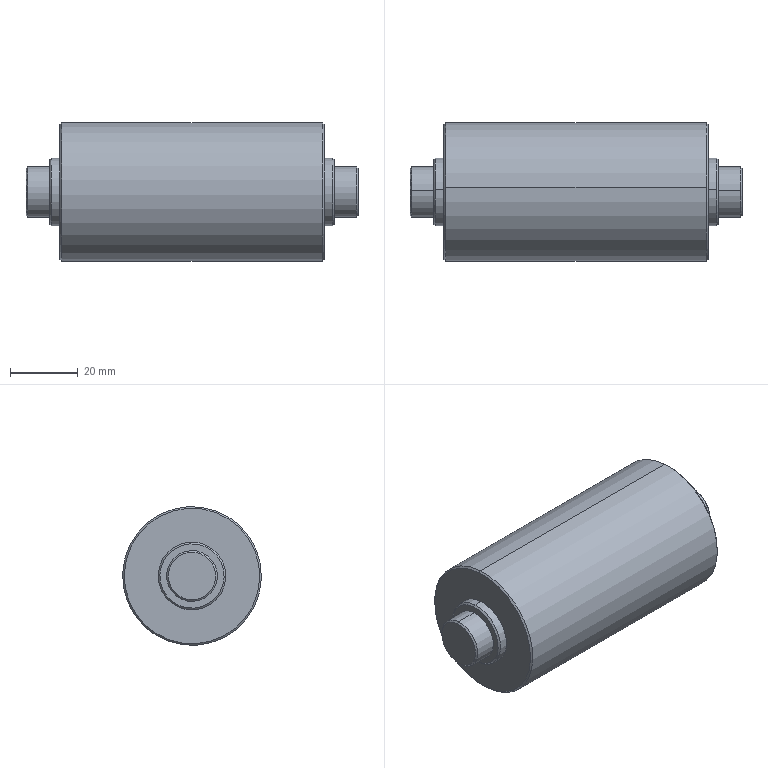Component | SolidWorks | ConveyorDrivenWheel-1 | 1 solid | 28 faces | box 98 x 41 x 41 mm | volume 107280 mm3 | cone 12 | cylinder 10 | plane 6 | commonest cylinder face diameters 15 x4 20 x4 41 x2 | material Plain Carbon Steel
build123d program:
from build123d import *

# Parameters (mm, degrees)
SKETCH1_R           = 20.5
BOSS_EXTRUDE1_DEPTH = 78
SKETCH2_R           = 10
BOSS_EXTRUDE2_DEPTH = 3
BOSS_EXTRUDE3_START = 3
SKETCH3_R           = 10
BOSS_EXTRUDE3_DEPTH = 3
SKETCH4_R           = 7.5
BOSS_EXTRUDE4_DEPTH = 7
BOSS_EXTRUDE5_START = 7
SKETCH5_R           = 7.5
BOSS_EXTRUDE5_DEPTH = 7
CHAMFER1_SIZE       = 0.5


with BuildPart() as part:
    # Sketch1 → Boss-Extrude1 (new body)
    with BuildSketch(Plane.XY):
        Circle(SKETCH1_R)
    extrude(amount=BOSS_EXTRUDE1_DEPTH)

    # Sketch2 → Boss-Extrude2 (add)
    with BuildSketch(Plane.XY.offset(78)):
        Circle(SKETCH2_R)
    extrude(amount=BOSS_EXTRUDE2_DEPTH)

    # Sketch3 → Boss-Extrude3 (add)
    with BuildSketch(Plane(origin=(0, 0, 0), x_dir=(-1, 0, 0), z_dir=(0, 0, -1)).offset(BOSS_EXTRUDE3_START)):
        with Locations(Location((0, 0, 0), (0, 0, 180))):
            Circle(SKETCH3_R)
    extrude(amount=-BOSS_EXTRUDE3_DEPTH)

    # Sketch4 → Boss-Extrude4 (add)
    with BuildSketch(Plane.XY.offset(81)):
        Circle(SKETCH4_R)
    extrude(amount=BOSS_EXTRUDE4_DEPTH)

    # Sketch5 → Boss-Extrude5 (add)
    with BuildSketch(Plane(origin=(0, 0, -3), x_dir=(-1, 0, 0), z_dir=(0, 0, -1)).offset(BOSS_EXTRUDE5_START)):
        with Locations(Location((0, 0, 0), (0, 0, 180))):
            Circle(SKETCH5_R)
    extrude(amount=-BOSS_EXTRUDE5_DEPTH)

    # Chamfer1
    chamfer1_edges = [part.edges().sort_by_distance(p)[0] for p in [
        (-10, 0, -3),
        (-7.5, 0, 88),
        (-20.5, 0, 0),
        (-7.5, 0, -10),
        (-20.5, 0, 78),
        (-10, 0, 81),
    ]]
    chamfer(chamfer1_edges, length=CHAMFER1_SIZE)


solid = part.part

# Placed as in the assembly
solid = solid.moved(Location((-44.55, 5.646, 155), (0, 90, 0)))
STEP:
#1=CARTESIAN_POINT('',(-1.754,0.2749,6.888));
#2=VERTEX_POINT('',#1);
#3=CARTESIAN_POINT('',(-1.754,0.1697,5.317));
#4=VERTEX_POINT('',#3);
#5=CARTESIAN_POINT('',(-1.754,0.2223,6.102));
#6=DIRECTION('',(-1.,0.,0.));
#7=DIRECTION('',(0.,0.06681,0.9978));
#8=AXIS2_PLACEMENT_3D('',#5,#6,#7);
#9=CIRCLE('',#8,0.7874);
#10=EDGE_CURVE('',#2,#4,#9,.T.);
#11=ORIENTED_EDGE('',*,*,#10,.F.);
#12=CARTESIAN_POINT('',(-1.734,0.2762,6.908));
#13=VERTEX_POINT('',#12);
#14=CARTESIAN_POINT('',(-1.754,0.2749,6.888));
#15=DIRECTION('',(0.7071,0.04724,0.7055));
#16=VECTOR('',#15,39.37);
#17=LINE('',#14,#16);
#18=EDGE_CURVE('',#2,#13,#17,.T.);
#19=ORIENTED_EDGE('',*,*,#18,.T.);
#20=CARTESIAN_POINT('',(-1.734,0.1684,5.297));
#21=VERTEX_POINT('',#20);
#22=CARTESIAN_POINT('',(-1.734,0.2223,6.102));
#23=DIRECTION('',(1.,0.,0.));
#24=DIRECTION('',(0.,0.06681,0.9978));
#25=AXIS2_PLACEMENT_3D('',#22,#23,#24);
#26=CIRCLE('',#25,0.8071);
#27=EDGE_CURVE('',#21,#13,#26,.T.);
#28=ORIENTED_EDGE('',*,*,#27,.F.);
#29=CARTESIAN_POINT('',(-1.754,0.1697,5.317));
#30=DIRECTION('',(0.7071,-0.04724,-0.7055));
#31=VECTOR('',#30,39.37);
#32=LINE('',#29,#31);
#33=EDGE_CURVE('',#4,#21,#32,.T.);
#34=ORIENTED_EDGE('',*,*,#33,.F.);
#35=EDGE_LOOP('',(#11,#19,#28,#34));
#36=FACE_OUTER_BOUND('',#35,.T.);
#37=CARTESIAN_POINT('',(-1.754,0.2223,6.102));
#38=DIRECTION('',(1.,0.,0.));
#39=DIRECTION('',(0.,-0.06681,-0.9978));
#40=AXIS2_PLACEMENT_3D('',#37,#38,#39);
#41=CONICAL_SURFACE('',#40,0.7874,0.7854);
#42=ADVANCED_FACE('',(#36),#41,.T.);
#43=CARTESIAN_POINT('',(1.317,0.1697,5.317));
#44=VERTEX_POINT('',#43);
#45=CARTESIAN_POINT('',(1.317,0.2749,6.888));
#46=VERTEX_POINT('',#45);
#47=CARTESIAN_POINT('',(1.317,0.2223,6.102));
#48=DIRECTION('',(1.,0.,0.));
#49=DIRECTION('',(0.,0.06681,0.9978));
#50=AXIS2_PLACEMENT_3D('',#47,#48,#49);
#51=CIRCLE('',#50,0.7874);
#52=EDGE_CURVE('',#44,#46,#51,.T.);
#53=ORIENTED_EDGE('',*,*,#52,.F.);
#54=CARTESIAN_POINT('',(1.297,0.1684,5.297));
#55=VERTEX_POINT('',#54);
#56=CARTESIAN_POINT('',(1.297,0.1684,5.297));
#57=DIRECTION('',(-0.7071,-0.04724,-0.7055));
#58=VECTOR('',#57,39.37);
#59=LINE('',#56,#58);
#60=EDGE_CURVE('',#44,#55,#59,.T.);
#61=ORIENTED_EDGE('',*,*,#60,.T.);
#62=CARTESIAN_POINT('',(1.297,0.2762,6.908));
#63=VERTEX_POINT('',#62);
#64=CARTESIAN_POINT('',(1.297,0.2223,6.102));
#65=DIRECTION('',(-1.,0.,0.));
#66=DIRECTION('',(0.,0.06681,0.9978));
#67=AXIS2_PLACEMENT_3D('',#64,#65,#66);
#68=CIRCLE('',#67,0.8071);
#69=EDGE_CURVE('',#63,#55,#68,.T.);
#70=ORIENTED_EDGE('',*,*,#69,.F.);
#71=CARTESIAN_POINT('',(1.297,0.2762,6.908));
#72=DIRECTION('',(-0.7071,0.04724,0.7055));
#73=VECTOR('',#72,39.37);
#74=LINE('',#71,#73);
#75=EDGE_CURVE('',#46,#63,#74,.T.);
#76=ORIENTED_EDGE('',*,*,#75,.F.);
#77=EDGE_LOOP('',(#53,#61,#70,#76));
#78=FACE_OUTER_BOUND('',#77,.T.);
#79=CARTESIAN_POINT('',(1.297,0.2223,6.102));
#80=DIRECTION('',(-1.,0.,0.));
#81=DIRECTION('',(0.,0.06681,0.9978));
#82=AXIS2_PLACEMENT_3D('',#79,#80,#81);
#83=CONICAL_SURFACE('',#82,0.8071,0.7854);
#84=ADVANCED_FACE('',(#78),#83,.T.);
#85=CARTESIAN_POINT('',(-2.148,0.2407,6.377));
#86=VERTEX_POINT('',#85);
#87=CARTESIAN_POINT('',(-2.148,0.2039,5.827));
#88=VERTEX_POINT('',#87);
#89=CARTESIAN_POINT('',(-2.148,0.2223,6.102));
#90=DIRECTION('',(-1.,0.,0.));
#91=DIRECTION('',(0.,0.06681,0.9978));
#92=AXIS2_PLACEMENT_3D('',#89,#90,#91);
#93=CIRCLE('',#92,0.2756);
#94=EDGE_CURVE('',#86,#88,#93,.T.);
#95=ORIENTED_EDGE('',*,*,#94,.F.);
#96=CARTESIAN_POINT('',(-2.128,0.242,6.397));
#97=VERTEX_POINT('',#96);
#98=CARTESIAN_POINT('',(-2.148,0.2407,6.377));
#99=DIRECTION('',(0.7071,0.04724,0.7055));
#100=VECTOR('',#99,39.37);
#101=LINE('',#98,#100);
#102=EDGE_CURVE('',#86,#97,#101,.T.);
#103=ORIENTED_EDGE('',*,*,#102,.T.);
#104=CARTESIAN_POINT('',(-2.128,0.2025,5.808));
#105=VERTEX_POINT('',#104);
#106=CARTESIAN_POINT('',(-2.128,0.2223,6.102));
#107=DIRECTION('',(1.,0.,0.));
#108=DIRECTION('',(0.,0.06681,0.9978));
#109=AXIS2_PLACEMENT_3D('',#106,#107,#108);
#110=CIRCLE('',#109,0.2953);
#111=EDGE_CURVE('',#105,#97,#110,.T.);
#112=ORIENTED_EDGE('',*,*,#111,.F.);
#113=CARTESIAN_POINT('',(-2.148,0.2039,5.827));
#114=DIRECTION('',(0.7071,-0.04724,-0.7055));
#115=VECTOR('',#114,39.37);
#116=LINE('',#113,#115);
#117=EDGE_CURVE('',#88,#105,#116,.T.);
#118=ORIENTED_EDGE('',*,*,#117,.F.);
#119=EDGE_LOOP('',(#95,#103,#112,#118));
#120=FACE_OUTER_BOUND('',#119,.T.);
#121=CARTESIAN_POINT('',(-2.148,0.2223,6.102));
#122=DIRECTION('',(1.,0.,0.));
#123=DIRECTION('',(0.,-0.06681,-0.9978));
#124=AXIS2_PLACEMENT_3D('',#121,#122,#123);
#125=CONICAL_SURFACE('',#124,0.2756,0.7854);
#126=ADVANCED_FACE('',(#120),#125,.T.);
#127=CARTESIAN_POINT('',(-1.872,0.2473,6.476));
#128=VERTEX_POINT('',#127);
#129=CARTESIAN_POINT('',(-1.872,0.1973,5.729));
#130=VERTEX_POINT('',#129);
#131=CARTESIAN_POINT('',(-1.872,0.2223,6.102));
#132=DIRECTION('',(-1.,0.,0.));
#133=DIRECTION('',(0.,0.06681,0.9978));
#134=AXIS2_PLACEMENT_3D('',#131,#132,#133);
#135=CIRCLE('',#134,0.374);
#136=EDGE_CURVE('',#128,#130,#135,.T.);
#137=ORIENTED_EDGE('',*,*,#136,.F.);
#138=CARTESIAN_POINT('',(-1.852,0.2486,6.495));
#139=VERTEX_POINT('',#138);
#140=CARTESIAN_POINT('',(-1.872,0.2473,6.476));
#141=DIRECTION('',(0.7071,0.04724,0.7055));
#142=VECTOR('',#141,39.37);
#143=LINE('',#140,#142);
#144=EDGE_CURVE('',#128,#139,#143,.T.);
#145=ORIENTED_EDGE('',*,*,#144,.T.);
#146=CARTESIAN_POINT('',(-1.852,0.196,5.71));
#147=VERTEX_POINT('',#146);
#148=CARTESIAN_POINT('',(-1.852,0.2223,6.102));
#149=DIRECTION('',(1.,0.,0.));
#150=DIRECTION('',(0.,0.06681,0.9978));
#151=AXIS2_PLACEMENT_3D('',#148,#149,#150);
#152=CIRCLE('',#151,0.3937);
#153=EDGE_CURVE('',#147,#139,#152,.T.);
#154=ORIENTED_EDGE('',*,*,#153,.F.);
#155=CARTESIAN_POINT('',(-1.872,0.1973,5.729));
#156=DIRECTION('',(0.7071,-0.04724,-0.7055));
#157=VECTOR('',#156,39.37);
#158=LINE('',#155,#157);
#159=EDGE_CURVE('',#130,#147,#158,.T.);
#160=ORIENTED_EDGE('',*,*,#159,.F.);
#161=EDGE_LOOP('',(#137,#145,#154,#160));
#162=FACE_OUTER_BOUND('',#161,.T.);
#163=CARTESIAN_POINT('',(-1.872,0.2223,6.102));
#164=DIRECTION('',(1.,0.,0.));
#165=DIRECTION('',(0.,-0.06681,-0.9978));
#166=AXIS2_PLACEMENT_3D('',#163,#164,#165);
#167=CONICAL_SURFACE('',#166,0.374,0.7854);
#168=ADVANCED_FACE('',(#162),#167,.T.);
#169=CARTESIAN_POINT('',(1.435,0.1973,5.729));
#170=VERTEX_POINT('',#169);
#171=CARTESIAN_POINT('',(1.435,0.2473,6.476));
#172=VERTEX_POINT('',#171);
#173=CARTESIAN_POINT('',(1.435,0.2223,6.102));
#174=DIRECTION('',(1.,0.,0.));
#175=DIRECTION('',(0.,-0.06681,-0.9978));
#176=AXIS2_PLACEMENT_3D('',#173,#174,#175);
#177=CIRCLE('',#176,0.374);
#178=EDGE_CURVE('',#170,#172,#177,.T.);
#179=ORIENTED_EDGE('',*,*,#178,.F.);
#180=CARTESIAN_POINT('',(1.415,0.196,5.71));
#181=VERTEX_POINT('',#180);
#182=CARTESIAN_POINT('',(1.435,0.1973,5.729));
#183=DIRECTION('',(-0.7071,-0.04724,-0.7055));
#184=VECTOR('',#183,39.37);
#185=LINE('',#182,#184);
#186=EDGE_CURVE('',#170,#181,#185,.T.);
#187=ORIENTED_EDGE('',*,*,#186,.T.);
#188=CARTESIAN_POINT('',(1.415,0.2486,6.495));
#189=VERTEX_POINT('',#188);
#190=CARTESIAN_POINT('',(1.415,0.2223,6.102));
#191=DIRECTION('',(-1.,0.,0.));
#192=DIRECTION('',(0.,-0.06681,-0.9978));
#193=AXIS2_PLACEMENT_3D('',#190,#191,#192);
#194=CIRCLE('',#193,0.3937);
#195=EDGE_CURVE('',#189,#181,#194,.T.);
#196=ORIENTED_EDGE('',*,*,#195,.F.);
#197=CARTESIAN_POINT('',(1.435,0.2473,6.476));
#198=DIRECTION('',(-0.7071,0.04724,0.7055));
#199=VECTOR('',#198,39.37);
#200=LINE('',#197,#199);
#201=EDGE_CURVE('',#172,#189,#200,.T.);
#202=ORIENTED_EDGE('',*,*,#201,.F.);
#203=EDGE_LOOP('',(#179,#187,#196,#202));
#204=FACE_OUTER_BOUND('',#203,.T.);
#205=CARTESIAN_POINT('',(1.435,0.2223,6.102));
#206=DIRECTION('',(-1.,0.,0.));
#207=DIRECTION('',(0.,0.06681,0.9978));
#208=AXIS2_PLACEMENT_3D('',#205,#206,#207);
#209=CONICAL_SURFACE('',#208,0.374,0.7854);
#210=ADVANCED_FACE('',(#204),#209,.T.);
#211=CARTESIAN_POINT('',(1.711,0.2039,5.827));
#212=VERTEX_POINT('',#211);
#213=CARTESIAN_POINT('',(1.711,0.2407,6.377));
#214=VERTEX_POINT('',#213);
#215=CARTESIAN_POINT('',(1.711,0.2223,6.102));
#216=DIRECTION('',(1.,0.,0.));
#217=DIRECTION('',(0.,-0.06681,-0.9978));
#218=AXIS2_PLACEMENT_3D('',#215,#216,#217);
#219=CIRCLE('',#218,0.2756);
#220=EDGE_CURVE('',#212,#214,#219,.T.);
#221=ORIENTED_EDGE('',*,*,#220,.F.);
#222=CARTESIAN_POINT('',(1.691,0.2025,5.808));
#223=VERTEX_POINT('',#222);
#224=CARTESIAN_POINT('',(1.711,0.2039,5.827));
#225=DIRECTION('',(-0.7071,-0.04724,-0.7055));
#226=VECTOR('',#225,39.37);
#227=LINE('',#224,#226);
#228=EDGE_CURVE('',#212,#223,#227,.T.);
#229=ORIENTED_EDGE('',*,*,#228,.T.);
#230=CARTESIAN_POINT('',(1.691,0.242,6.397));
#231=VERTEX_POINT('',#230);
#232=CARTESIAN_POINT('',(1.691,0.2223,6.102));
#233=DIRECTION('',(-1.,0.,0.));
#234=DIRECTION('',(0.,-0.06681,-0.9978));
#235=AXIS2_PLACEMENT_3D('',#232,#233,#234);
#236=CIRCLE('',#235,0.2953);
#237=EDGE_CURVE('',#231,#223,#236,.T.);
#238=ORIENTED_EDGE('',*,*,#237,.F.);
#239=CARTESIAN_POINT('',(1.711,0.2407,6.377));
#240=DIRECTION('',(-0.7071,0.04724,0.7055));
#241=VECTOR('',#240,39.37);
#242=LINE('',#239,#241);
#243=EDGE_CURVE('',#214,#231,#242,.T.);
#244=ORIENTED_EDGE('',*,*,#243,.F.);
#245=EDGE_LOOP('',(#221,#229,#238,#244));
#246=FACE_OUTER_BOUND('',#245,.T.);
#247=CARTESIAN_POINT('',(1.711,0.2223,6.102));
#248=DIRECTION('',(-1.,0.,0.));
#249=DIRECTION('',(0.,0.06681,0.9978));
#250=AXIS2_PLACEMENT_3D('',#247,#248,#249);
#251=CONICAL_SURFACE('',#250,0.2756,0.7854);
#252=ADVANCED_FACE('',(#246),#251,.T.);
#253=ORIENTED_EDGE('',*,*,#237,.T.);
#254=CARTESIAN_POINT('',(1.435,0.2025,5.808));
#255=VERTEX_POINT('',#254);
#256=CARTESIAN_POINT('',(1.711,0.2025,5.808));
#257=DIRECTION('',(-1.,0.,0.));
#258=VECTOR('',#257,39.37);
#259=LINE('',#256,#258);
#260=EDGE_CURVE('',#223,#255,#259,.T.);
#261=ORIENTED_EDGE('',*,*,#260,.T.);
#262=CARTESIAN_POINT('',(1.435,0.242,6.397));
#263=VERTEX_POINT('',#262);
#264=CARTESIAN_POINT('',(1.435,0.2223,6.102));
#265=DIRECTION('',(1.,0.,0.));
#266=DIRECTION('',(0.,-0.06681,-0.9978));
#267=AXIS2_PLACEMENT_3D('',#264,#265,#266);
#268=CIRCLE('',#267,0.2953);
#269=EDGE_CURVE('',#255,#263,#268,.T.);
#270=ORIENTED_EDGE('',*,*,#269,.T.);
#271=CARTESIAN_POINT('',(1.711,0.242,6.397));
#272=DIRECTION('',(-1.,0.,0.));
#273=VECTOR('',#272,39.37);
#274=LINE('',#271,#273);
#275=EDGE_CURVE('',#231,#263,#274,.T.);
#276=ORIENTED_EDGE('',*,*,#275,.F.);
#277=EDGE_LOOP('',(#253,#261,#270,#276));
#278=FACE_OUTER_BOUND('',#277,.T.);
#279=CARTESIAN_POINT('',(1.711,0.2223,6.102));
#280=DIRECTION('',(-1.,0.,0.));
#281=DIRECTION('',(0.,0.06681,0.9978));
#282=AXIS2_PLACEMENT_3D('',#279,#280,#281);
#283=CYLINDRICAL_SURFACE('',#282,0.2953);
#284=ADVANCED_FACE('',(#278),#283,.T.);
#285=ORIENTED_EDGE('',*,*,#111,.T.);
#286=CARTESIAN_POINT('',(-1.872,0.242,6.397));
#287=VERTEX_POINT('',#286);
#288=CARTESIAN_POINT('',(-2.148,0.242,6.397));
#289=DIRECTION('',(1.,0.,0.));
#290=VECTOR('',#289,39.37);
#291=LINE('',#288,#290);
#292=EDGE_CURVE('',#97,#287,#291,.T.);
#293=ORIENTED_EDGE('',*,*,#292,.T.);
#294=CARTESIAN_POINT('',(-1.872,0.2025,5.808));
#295=VERTEX_POINT('',#294);
#296=CARTESIAN_POINT('',(-1.872,0.2223,6.102));
#297=DIRECTION('',(-1.,0.,0.));
#298=DIRECTION('',(0.,0.06681,0.9978));
#299=AXIS2_PLACEMENT_3D('',#296,#297,#298);
#300=CIRCLE('',#299,0.2953);
#301=EDGE_CURVE('',#287,#295,#300,.T.);
#302=ORIENTED_EDGE('',*,*,#301,.T.);
#303=CARTESIAN_POINT('',(-2.148,0.2025,5.808));
#304=DIRECTION('',(1.,0.,0.));
#305=VECTOR('',#304,39.37);
#306=LINE('',#303,#305);
#307=EDGE_CURVE('',#105,#295,#306,.T.);
#308=ORIENTED_EDGE('',*,*,#307,.F.);
#309=EDGE_LOOP('',(#285,#293,#302,#308));
#310=FACE_OUTER_BOUND('',#309,.T.);
#311=CARTESIAN_POINT('',(-2.148,0.2223,6.102));
#312=DIRECTION('',(1.,0.,0.));
#313=DIRECTION('',(0.,-0.06681,-0.9978));
#314=AXIS2_PLACEMENT_3D('',#311,#312,#313);
#315=CYLINDRICAL_SURFACE('',#314,0.2953);
#316=ADVANCED_FACE('',(#310),#315,.T.);
#317=ORIENTED_EDGE('',*,*,#195,.T.);
#318=CARTESIAN_POINT('',(1.317,0.196,5.71));
#319=VERTEX_POINT('',#318);
#320=CARTESIAN_POINT('',(1.435,0.196,5.71));
#321=DIRECTION('',(-1.,0.,0.));
#322=VECTOR('',#321,39.37);
#323=LINE('',#320,#322);
#324=EDGE_CURVE('',#181,#319,#323,.T.);
#325=ORIENTED_EDGE('',*,*,#324,.T.);
#326=CARTESIAN_POINT('',(1.317,0.2486,6.495));
#327=VERTEX_POINT('',#326);
#328=CARTESIAN_POINT('',(1.317,0.2223,6.102));
#329=DIRECTION('',(1.,0.,0.));
#330=DIRECTION('',(0.,0.06681,0.9978));
#331=AXIS2_PLACEMENT_3D('',#328,#329,#330);
#332=CIRCLE('',#331,0.3937);
#333=EDGE_CURVE('',#319,#327,#332,.T.);
#334=ORIENTED_EDGE('',*,*,#333,.T.);
#335=CARTESIAN_POINT('',(1.435,0.2486,6.495));
#336=DIRECTION('',(-1.,0.,0.));
#337=VECTOR('',#336,39.37);
#338=LINE('',#335,#337);
#339=EDGE_CURVE('',#189,#327,#338,.T.);
#340=ORIENTED_EDGE('',*,*,#339,.F.);
#341=EDGE_LOOP('',(#317,#325,#334,#340));
#342=FACE_OUTER_BOUND('',#341,.T.);
#343=CARTESIAN_POINT('',(1.435,0.2223,6.102));
#344=DIRECTION('',(-1.,0.,0.));
#345=DIRECTION('',(0.,0.06681,0.9978));
#346=AXIS2_PLACEMENT_3D('',#343,#344,#345);
#347=CYLINDRICAL_SURFACE('',#346,0.3937);
#348=ADVANCED_FACE('',(#342),#347,.T.);
#349=ORIENTED_EDGE('',*,*,#153,.T.);
#350=CARTESIAN_POINT('',(-1.754,0.2486,6.495));
#351=VERTEX_POINT('',#350);
#352=CARTESIAN_POINT('',(-1.872,0.2486,6.495));
#353=DIRECTION('',(1.,0.,0.));
#354=VECTOR('',#353,39.37);
#355=LINE('',#352,#354);
#356=EDGE_CURVE('',#139,#351,#355,.T.);
#357=ORIENTED_EDGE('',*,*,#356,.T.);
#358=CARTESIAN_POINT('',(-1.754,0.196,5.71));
#359=VERTEX_POINT('',#358);
#360=CARTESIAN_POINT('',(-1.754,0.2223,6.102));
#361=DIRECTION('',(-1.,0.,0.));
#362=DIRECTION('',(0.,0.06681,0.9978));
#363=AXIS2_PLACEMENT_3D('',#360,#361,#362);
#364=CIRCLE('',#363,0.3937);
#365=EDGE_CURVE('',#351,#359,#364,.T.);
#366=ORIENTED_EDGE('',*,*,#365,.T.);
#367=CARTESIAN_POINT('',(-1.872,0.196,5.71));
#368=DIRECTION('',(1.,0.,0.));
#369=VECTOR('',#368,39.37);
#370=LINE('',#367,#369);
#371=EDGE_CURVE('',#147,#359,#370,.T.);
#372=ORIENTED_EDGE('',*,*,#371,.F.);
#373=EDGE_LOOP('',(#349,#357,#366,#372));
#374=FACE_OUTER_BOUND('',#373,.T.);
#375=CARTESIAN_POINT('',(-1.872,0.2223,6.102));
#376=DIRECTION('',(1.,0.,0.));
#377=DIRECTION('',(0.,-0.06681,-0.9978));
#378=AXIS2_PLACEMENT_3D('',#375,#376,#377);
#379=CYLINDRICAL_SURFACE('',#378,0.3937);
#380=ADVANCED_FACE('',(#374),#379,.T.);
#381=ORIENTED_EDGE('',*,*,#27,.T.);
#382=CARTESIAN_POINT('',(-1.754,0.2762,6.908));
#383=DIRECTION('',(1.,0.,0.));
#384=VECTOR('',#383,39.37);
#385=LINE('',#382,#384);
#386=EDGE_CURVE('',#13,#63,#385,.T.);
#387=ORIENTED_EDGE('',*,*,#386,.T.);
#388=ORIENTED_EDGE('',*,*,#69,.T.);
#389=CARTESIAN_POINT('',(-1.754,0.1684,5.297));
#390=DIRECTION('',(1.,0.,0.));
#391=VECTOR('',#390,39.37);
#392=LINE('',#389,#391);
#393=EDGE_CURVE('',#21,#55,#392,.T.);
#394=ORIENTED_EDGE('',*,*,#393,.F.);
#395=EDGE_LOOP('',(#381,#387,#388,#394));
#396=FACE_OUTER_BOUND('',#395,.T.);
#397=CARTESIAN_POINT('',(-1.754,0.2223,6.102));
#398=DIRECTION('',(1.,0.,0.));
#399=DIRECTION('',(0.,-0.06681,-0.9978));
#400=AXIS2_PLACEMENT_3D('',#397,#398,#399);
#401=CYLINDRICAL_SURFACE('',#400,0.8071);
#402=ADVANCED_FACE('',(#396),#401,.T.);
#403=CARTESIAN_POINT('',(1.435,0.2223,6.102));
#404=DIRECTION('',(1.,0.,0.));
#405=DIRECTION('',(0.,-0.06681,-0.9978));
#406=AXIS2_PLACEMENT_3D('',#403,#404,#405);
#407=CIRCLE('',#406,0.374);
#408=EDGE_CURVE('',#172,#170,#407,.T.);
#409=ORIENTED_EDGE('',*,*,#408,.T.);
#410=ORIENTED_EDGE('',*,*,#178,.T.);
#411=EDGE_LOOP('',(#409,#410));
#412=FACE_OUTER_BOUND('',#411,.T.);
#413=CARTESIAN_POINT('',(1.435,0.2223,6.102));
#414=DIRECTION('',(1.,0.,0.));
#415=DIRECTION('',(0.,-0.06681,-0.9978));
#416=AXIS2_PLACEMENT_3D('',#413,#414,#415);
#417=CIRCLE('',#416,0.2953);
#418=EDGE_CURVE('',#263,#255,#417,.T.);
#419=ORIENTED_EDGE('',*,*,#418,.F.);
#420=ORIENTED_EDGE('',*,*,#269,.F.);
#421=EDGE_LOOP('',(#419,#420));
#422=FACE_BOUND('',#421,.T.);
#423=CARTESIAN_POINT('',(1.435,0.2223,6.102));
#424=DIRECTION('',(1.,0.,0.));
#425=DIRECTION('',(0.,-0.06681,-0.9978));
#426=AXIS2_PLACEMENT_3D('',#423,#424,#425);
#427=PLANE('',#426);
#428=ADVANCED_FACE('',(#412,#422),#427,.T.);
#429=CARTESIAN_POINT('',(-1.872,0.2223,6.102));
#430=DIRECTION('',(-1.,0.,0.));
#431=DIRECTION('',(0.,0.06681,0.9978));
#432=AXIS2_PLACEMENT_3D('',#429,#430,#431);
#433=CIRCLE('',#432,0.374);
#434=EDGE_CURVE('',#130,#128,#433,.T.);
#435=ORIENTED_EDGE('',*,*,#434,.T.);
#436=ORIENTED_EDGE('',*,*,#136,.T.);
#437=EDGE_LOOP('',(#435,#436));
#438=FACE_OUTER_BOUND('',#437,.T.);
#439=CARTESIAN_POINT('',(-1.872,0.2223,6.102));
#440=DIRECTION('',(-1.,0.,0.));
#441=DIRECTION('',(0.,0.06681,0.9978));
#442=AXIS2_PLACEMENT_3D('',#439,#440,#441);
#443=CIRCLE('',#442,0.2953);
#444=EDGE_CURVE('',#295,#287,#443,.T.);
#445=ORIENTED_EDGE('',*,*,#444,.F.);
#446=ORIENTED_EDGE('',*,*,#301,.F.);
#447=EDGE_LOOP('',(#445,#446));
#448=FACE_BOUND('',#447,.T.);
#449=CARTESIAN_POINT('',(-1.872,0.2223,6.102));
#450=DIRECTION('',(-1.,0.,0.));
#451=DIRECTION('',(0.,0.06681,0.9978));
#452=AXIS2_PLACEMENT_3D('',#449,#450,#451);
#453=PLANE('',#452);
#454=ADVANCED_FACE('',(#438,#448),#453,.T.);
#455=CARTESIAN_POINT('',(1.317,0.2223,6.102));
#456=DIRECTION('',(1.,0.,0.));
#457=DIRECTION('',(0.,0.06681,0.9978));
#458=AXIS2_PLACEMENT_3D('',#455,#456,#457);
#459=CIRCLE('',#458,0.7874);
#460=EDGE_CURVE('',#46,#44,#459,.T.);
#461=ORIENTED_EDGE('',*,*,#460,.T.);
#462=ORIENTED_EDGE('',*,*,#52,.T.);
#463=EDGE_LOOP('',(#461,#462));
#464=FACE_OUTER_BOUND('',#463,.T.);
#465=CARTESIAN_POINT('',(1.317,0.2223,6.102));
#466=DIRECTION('',(1.,0.,0.));
#467=DIRECTION('',(0.,0.06681,0.9978));
#468=AXIS2_PLACEMENT_3D('',#465,#466,#467);
#469=CIRCLE('',#468,0.3937);
#470=EDGE_CURVE('',#327,#319,#469,.T.);
#471=ORIENTED_EDGE('',*,*,#470,.F.);
#472=ORIENTED_EDGE('',*,*,#333,.F.);
#473=EDGE_LOOP('',(#471,#472));
#474=FACE_BOUND('',#473,.T.);
#475=CARTESIAN_POINT('',(1.317,0.2223,6.102));
#476=DIRECTION('',(-1.,0.,0.));
#477=DIRECTION('',(0.,0.06681,0.9978));
#478=AXIS2_PLACEMENT_3D('',#475,#476,#477);
#479=PLANE('',#478);
#480=ADVANCED_FACE('',(#464,#474),#479,.F.);
#481=CARTESIAN_POINT('',(-1.754,0.2223,6.102));
#482=DIRECTION('',(-1.,0.,0.));
#483=DIRECTION('',(0.,0.06681,0.9978));
#484=AXIS2_PLACEMENT_3D('',#481,#482,#483);
#485=CIRCLE('',#484,0.7874);
#486=EDGE_CURVE('',#4,#2,#485,.T.);
#487=ORIENTED_EDGE('',*,*,#486,.T.);
#488=ORIENTED_EDGE('',*,*,#10,.T.);
#489=EDGE_LOOP('',(#487,#488));
#490=FACE_OUTER_BOUND('',#489,.T.);
#491=CARTESIAN_POINT('',(-1.754,0.2223,6.102));
#492=DIRECTION('',(-1.,0.,0.));
#493=DIRECTION('',(0.,0.06681,0.9978));
#494=AXIS2_PLACEMENT_3D('',#491,#492,#493);
#495=CIRCLE('',#494,0.3937);
#496=EDGE_CURVE('',#359,#351,#495,.T.);
#497=ORIENTED_EDGE('',*,*,#496,.F.);
#498=ORIENTED_EDGE('',*,*,#365,.F.);
#499=EDGE_LOOP('',(#497,#498));
#500=FACE_BOUND('',#499,.T.);
#501=CARTESIAN_POINT('',(-1.754,0.2223,6.102));
#502=DIRECTION('',(-1.,0.,0.));
#503=DIRECTION('',(0.,0.06681,0.9978));
#504=AXIS2_PLACEMENT_3D('',#501,#502,#503);
#505=PLANE('',#504);
#506=ADVANCED_FACE('',(#490,#500),#505,.T.);
#507=ORIENTED_EDGE('',*,*,#386,.F.);
#508=CARTESIAN_POINT('',(-1.734,0.2223,6.102));
#509=DIRECTION('',(1.,0.,0.));
#510=DIRECTION('',(0.,0.06681,0.9978));
#511=AXIS2_PLACEMENT_3D('',#508,#509,#510);
#512=CIRCLE('',#511,0.8071);
#513=EDGE_CURVE('',#13,#21,#512,.T.);
#514=ORIENTED_EDGE('',*,*,#513,.T.);
#515=ORIENTED_EDGE('',*,*,#393,.T.);
#516=CARTESIAN_POINT('',(1.297,0.2223,6.102));
#517=DIRECTION('',(-1.,0.,0.));
#518=DIRECTION('',(0.,0.06681,0.9978));
#519=AXIS2_PLACEMENT_3D('',#516,#517,#518);
#520=CIRCLE('',#519,0.8071);
#521=EDGE_CURVE('',#55,#63,#520,.T.);
#522=ORIENTED_EDGE('',*,*,#521,.T.);
#523=EDGE_LOOP('',(#507,#514,#515,#522));
#524=FACE_OUTER_BOUND('',#523,.T.);
#525=CARTESIAN_POINT('',(-1.754,0.2223,6.102));
#526=DIRECTION('',(1.,0.,0.));
#527=DIRECTION('',(0.,-0.06681,-0.9978));
#528=AXIS2_PLACEMENT_3D('',#525,#526,#527);
#529=CYLINDRICAL_SURFACE('',#528,0.8071);
#530=ADVANCED_FACE('',(#524),#529,.T.);
#531=ORIENTED_EDGE('',*,*,#356,.F.);
#532=CARTESIAN_POINT('',(-1.852,0.2223,6.102));
#533=DIRECTION('',(1.,0.,0.));
#534=DIRECTION('',(0.,0.06681,0.9978));
#535=AXIS2_PLACEMENT_3D('',#532,#533,#534);
#536=CIRCLE('',#535,0.3937);
#537=EDGE_CURVE('',#139,#147,#536,.T.);
#538=ORIENTED_EDGE('',*,*,#537,.T.);
#539=ORIENTED_EDGE('',*,*,#371,.T.);
#540=ORIENTED_EDGE('',*,*,#496,.T.);
#541=EDGE_LOOP('',(#531,#538,#539,#540));
#542=FACE_OUTER_BOUND('',#541,.T.);
#543=CARTESIAN_POINT('',(-1.872,0.2223,6.102));
#544=DIRECTION('',(1.,0.,0.));
#545=DIRECTION('',(0.,-0.06681,-0.9978));
#546=AXIS2_PLACEMENT_3D('',#543,#544,#545);
#547=CYLINDRICAL_SURFACE('',#546,0.3937);
#548=ADVANCED_FACE('',(#542),#547,.T.);
#549=ORIENTED_EDGE('',*,*,#324,.F.);
#550=CARTESIAN_POINT('',(1.415,0.2223,6.102));
#551=DIRECTION('',(-1.,0.,0.));
#552=DIRECTION('',(0.,-0.06681,-0.9978));
#553=AXIS2_PLACEMENT_3D('',#550,#551,#552);
#554=CIRCLE('',#553,0.3937);
#555=EDGE_CURVE('',#181,#189,#554,.T.);
#556=ORIENTED_EDGE('',*,*,#555,.T.);
#557=ORIENTED_EDGE('',*,*,#339,.T.);
#558=ORIENTED_EDGE('',*,*,#470,.T.);
#559=EDGE_LOOP('',(#549,#556,#557,#558));
#560=FACE_OUTER_BOUND('',#559,.T.);
#561=CARTESIAN_POINT('',(1.435,0.2223,6.102));
#562=DIRECTION('',(-1.,0.,0.));
#563=DIRECTION('',(0.,0.06681,0.9978));
#564=AXIS2_PLACEMENT_3D('',#561,#562,#563);
#565=CYLINDRICAL_SURFACE('',#564,0.3937);
#566=ADVANCED_FACE('',(#560),#565,.T.);
#567=ORIENTED_EDGE('',*,*,#292,.F.);
#568=CARTESIAN_POINT('',(-2.128,0.2223,6.102));
#569=DIRECTION('',(1.,0.,0.));
#570=DIRECTION('',(0.,0.06681,0.9978));
#571=AXIS2_PLACEMENT_3D('',#568,#569,#570);
#572=CIRCLE('',#571,0.2953);
#573=EDGE_CURVE('',#97,#105,#572,.T.);
#574=ORIENTED_EDGE('',*,*,#573,.T.);
#575=ORIENTED_EDGE('',*,*,#307,.T.);
#576=ORIENTED_EDGE('',*,*,#444,.T.);
#577=EDGE_LOOP('',(#567,#574,#575,#576));
#578=FACE_OUTER_BOUND('',#577,.T.);
#579=CARTESIAN_POINT('',(-2.148,0.2223,6.102));
#580=DIRECTION('',(1.,0.,0.));
#581=DIRECTION('',(0.,-0.06681,-0.9978));
#582=AXIS2_PLACEMENT_3D('',#579,#580,#581);
#583=CYLINDRICAL_SURFACE('',#582,0.2953);
#584=ADVANCED_FACE('',(#578),#583,.T.);
#585=CARTESIAN_POINT('',(-2.148,0.2223,6.102));
#586=DIRECTION('',(-1.,0.,0.));
#587=DIRECTION('',(0.,0.06681,0.9978));
#588=AXIS2_PLACEMENT_3D('',#585,#586,#587);
#589=CIRCLE('',#588,0.2756);
#590=EDGE_CURVE('',#88,#86,#589,.T.);
#591=ORIENTED_EDGE('',*,*,#590,.T.);
#592=ORIENTED_EDGE('',*,*,#94,.T.);
#593=EDGE_LOOP('',(#591,#592));
#594=FACE_OUTER_BOUND('',#593,.T.);
#595=CARTESIAN_POINT('',(-2.148,0.2223,6.102));
#596=DIRECTION('',(-1.,0.,0.));
#597=DIRECTION('',(0.,0.06681,0.9978));
#598=AXIS2_PLACEMENT_3D('',#595,#596,#597);
#599=PLANE('',#598);
#600=ADVANCED_FACE('',(#594),#599,.T.);
#601=ORIENTED_EDGE('',*,*,#260,.F.);
#602=CARTESIAN_POINT('',(1.691,0.2223,6.102));
#603=DIRECTION('',(-1.,0.,0.));
#604=DIRECTION('',(0.,-0.06681,-0.9978));
#605=AXIS2_PLACEMENT_3D('',#602,#603,#604);
#606=CIRCLE('',#605,0.2953);
#607=EDGE_CURVE('',#223,#231,#606,.T.);
#608=ORIENTED_EDGE('',*,*,#607,.T.);
#609=ORIENTED_EDGE('',*,*,#275,.T.);
#610=ORIENTED_EDGE('',*,*,#418,.T.);
#611=EDGE_LOOP('',(#601,#608,#609,#610));
#612=FACE_OUTER_BOUND('',#611,.T.);
#613=CARTESIAN_POINT('',(1.711,0.2223,6.102));
#614=DIRECTION('',(-1.,0.,0.));
#615=DIRECTION('',(0.,0.06681,0.9978));
#616=AXIS2_PLACEMENT_3D('',#613,#614,#615);
#617=CYLINDRICAL_SURFACE('',#616,0.2953);
#618=ADVANCED_FACE('',(#612),#617,.T.);
#619=CARTESIAN_POINT('',(1.711,0.2223,6.102));
#620=DIRECTION('',(1.,0.,0.));
#621=DIRECTION('',(0.,-0.06681,-0.9978));
#622=AXIS2_PLACEMENT_3D('',#619,#620,#621);
#623=CIRCLE('',#622,0.2756);
#624=EDGE_CURVE('',#214,#212,#623,.T.);
#625=ORIENTED_EDGE('',*,*,#624,.T.);
#626=ORIENTED_EDGE('',*,*,#220,.T.);
#627=EDGE_LOOP('',(#625,#626));
#628=FACE_OUTER_BOUND('',#627,.T.);
#629=CARTESIAN_POINT('',(1.711,0.2223,6.102));
#630=DIRECTION('',(1.,0.,0.));
#631=DIRECTION('',(0.,-0.06681,-0.9978));
#632=AXIS2_PLACEMENT_3D('',#629,#630,#631);
#633=PLANE('',#632);
#634=ADVANCED_FACE('',(#628),#633,.T.);
#635=ORIENTED_EDGE('',*,*,#228,.F.);
#636=ORIENTED_EDGE('',*,*,#624,.F.);
#637=ORIENTED_EDGE('',*,*,#243,.T.);
#638=ORIENTED_EDGE('',*,*,#607,.F.);
#639=EDGE_LOOP('',(#635,#636,#637,#638));
#640=FACE_OUTER_BOUND('',#639,.T.);
#641=CARTESIAN_POINT('',(1.711,0.2223,6.102));
#642=DIRECTION('',(-1.,0.,0.));
#643=DIRECTION('',(0.,0.06681,0.9978));
#644=AXIS2_PLACEMENT_3D('',#641,#642,#643);
#645=CONICAL_SURFACE('',#644,0.2756,0.7854);
#646=ADVANCED_FACE('',(#640),#645,.T.);
#647=ORIENTED_EDGE('',*,*,#186,.F.);
#648=ORIENTED_EDGE('',*,*,#408,.F.);
#649=ORIENTED_EDGE('',*,*,#201,.T.);
#650=ORIENTED_EDGE('',*,*,#555,.F.);
#651=EDGE_LOOP('',(#647,#648,#649,#650));
#652=FACE_OUTER_BOUND('',#651,.T.);
#653=CARTESIAN_POINT('',(1.435,0.2223,6.102));
#654=DIRECTION('',(-1.,0.,0.));
#655=DIRECTION('',(0.,0.06681,0.9978));
#656=AXIS2_PLACEMENT_3D('',#653,#654,#655);
#657=CONICAL_SURFACE('',#656,0.374,0.7854);
#658=ADVANCED_FACE('',(#652),#657,.T.);
#659=ORIENTED_EDGE('',*,*,#144,.F.);
#660=ORIENTED_EDGE('',*,*,#434,.F.);
#661=ORIENTED_EDGE('',*,*,#159,.T.);
#662=ORIENTED_EDGE('',*,*,#537,.F.);
#663=EDGE_LOOP('',(#659,#660,#661,#662));
#664=FACE_OUTER_BOUND('',#663,.T.);
#665=CARTESIAN_POINT('',(-1.872,0.2223,6.102));
#666=DIRECTION('',(1.,0.,0.));
#667=DIRECTION('',(0.,-0.06681,-0.9978));
#668=AXIS2_PLACEMENT_3D('',#665,#666,#667);
#669=CONICAL_SURFACE('',#668,0.374,0.7854);
#670=ADVANCED_FACE('',(#664),#669,.T.);
#671=ORIENTED_EDGE('',*,*,#102,.F.);
#672=ORIENTED_EDGE('',*,*,#590,.F.);
#673=ORIENTED_EDGE('',*,*,#117,.T.);
#674=ORIENTED_EDGE('',*,*,#573,.F.);
#675=EDGE_LOOP('',(#671,#672,#673,#674));
#676=FACE_OUTER_BOUND('',#675,.T.);
#677=CARTESIAN_POINT('',(-2.148,0.2223,6.102));
#678=DIRECTION('',(1.,0.,0.));
#679=DIRECTION('',(0.,-0.06681,-0.9978));
#680=AXIS2_PLACEMENT_3D('',#677,#678,#679);
#681=CONICAL_SURFACE('',#680,0.2756,0.7854);
#682=ADVANCED_FACE('',(#676),#681,.T.);
#683=ORIENTED_EDGE('',*,*,#60,.F.);
#684=ORIENTED_EDGE('',*,*,#460,.F.);
#685=ORIENTED_EDGE('',*,*,#75,.T.);
#686=ORIENTED_EDGE('',*,*,#521,.F.);
#687=EDGE_LOOP('',(#683,#684,#685,#686));
#688=FACE_OUTER_BOUND('',#687,.T.);
#689=CARTESIAN_POINT('',(1.297,0.2223,6.102));
#690=DIRECTION('',(-1.,0.,0.));
#691=DIRECTION('',(0.,0.06681,0.9978));
#692=AXIS2_PLACEMENT_3D('',#689,#690,#691);
#693=CONICAL_SURFACE('',#692,0.8071,0.7854);
#694=ADVANCED_FACE('',(#688),#693,.T.);
#695=ORIENTED_EDGE('',*,*,#18,.F.);
#696=ORIENTED_EDGE('',*,*,#486,.F.);
#697=ORIENTED_EDGE('',*,*,#33,.T.);
#698=ORIENTED_EDGE('',*,*,#513,.F.);
#699=EDGE_LOOP('',(#695,#696,#697,#698));
#700=FACE_OUTER_BOUND('',#699,.T.);
#701=CARTESIAN_POINT('',(-1.754,0.2223,6.102));
#702=DIRECTION('',(1.,0.,0.));
#703=DIRECTION('',(0.,-0.06681,-0.9978));
#704=AXIS2_PLACEMENT_3D('',#701,#702,#703);
#705=CONICAL_SURFACE('',#704,0.7874,0.7854);
#706=ADVANCED_FACE('',(#700),#705,.T.);
#707=CLOSED_SHELL('',(#42,#84,#126,#168,#210,#252,#284,#316,#348,#380,#402,#428,#454,#480,#506,#530,#548,#566,#584,#600,#618,#634,#646,#658,#670,#682,#694,#706));
#708=MANIFOLD_SOLID_BREP('',#707);
#709=CARTESIAN_POINT('',(0.,0.,0.));
#710=DIRECTION('',(0.,0.,1.));
#711=DIRECTION('',(1.,0.,0.));
#712=AXIS2_PLACEMENT_3D('',#709,#710,#711);
#713=(LENGTH_UNIT()NAMED_UNIT(*)SI_UNIT($,.METRE.));
#714=LENGTH_MEASURE_WITH_UNIT(LENGTH_MEASURE(0.0254),#713);
#715=DIMENSIONAL_EXPONENTS(1.,0.,0.,0.,0.,0.,0.);
#716=(CONVERSION_BASED_UNIT('',#714)LENGTH_UNIT()NAMED_UNIT(#715));
#717=UNCERTAINTY_MEASURE_WITH_UNIT(LENGTH_MEASURE(0.00001),#716,'','');
#718=(NAMED_UNIT(*)PLANE_ANGLE_UNIT()SI_UNIT($,.RADIAN.));
#719=(NAMED_UNIT(*)SI_UNIT($,.STERADIAN.)SOLID_ANGLE_UNIT());
#720=(GEOMETRIC_REPRESENTATION_CONTEXT(3)GLOBAL_UNCERTAINTY_ASSIGNED_CONTEXT((#717))GLOBAL_UNIT_ASSIGNED_CONTEXT((#716,#718,#719))REPRESENTATION_CONTEXT('',''));
#721=ADVANCED_BREP_SHAPE_REPRESENTATION('',(#708,#712),#720);
#722=COLOUR_RGB('',0.7922,0.8196,0.9333);
#723=FILL_AREA_STYLE_COLOUR('',#722);
#724=FILL_AREA_STYLE('',(#723));
#725=SURFACE_STYLE_FILL_AREA(#724);
#726=SURFACE_SIDE_STYLE('',(#725));
#727=SURFACE_STYLE_USAGE(.BOTH.,#726);
#728=PRESENTATION_STYLE_ASSIGNMENT((#727));
#729=STYLED_ITEM('',(#728),#708);
#730=(LENGTH_UNIT()NAMED_UNIT(*)SI_UNIT($,.METRE.));
#731=LENGTH_MEASURE_WITH_UNIT(LENGTH_MEASURE(0.0254),#730);
#732=DIMENSIONAL_EXPONENTS(1.,0.,0.,0.,0.,0.,0.);
#733=(CONVERSION_BASED_UNIT('',#731)LENGTH_UNIT()NAMED_UNIT(#732));
#734=UNCERTAINTY_MEASURE_WITH_UNIT(LENGTH_MEASURE(0.00001),#733,'','');
#735=(NAMED_UNIT(*)PLANE_ANGLE_UNIT()SI_UNIT($,.RADIAN.));
#736=(NAMED_UNIT(*)SI_UNIT($,.STERADIAN.)SOLID_ANGLE_UNIT());
#737=(GEOMETRIC_REPRESENTATION_CONTEXT(3)GLOBAL_UNCERTAINTY_ASSIGNED_CONTEXT((#734))GLOBAL_UNIT_ASSIGNED_CONTEXT((#733,#735,#736))REPRESENTATION_CONTEXT('',''));
#738=MECHANICAL_DESIGN_GEOMETRIC_PRESENTATION_REPRESENTATION('',(#729),#737);
#739=PRESENTATION_LAYER_ASSIGNMENT('','',(#729));